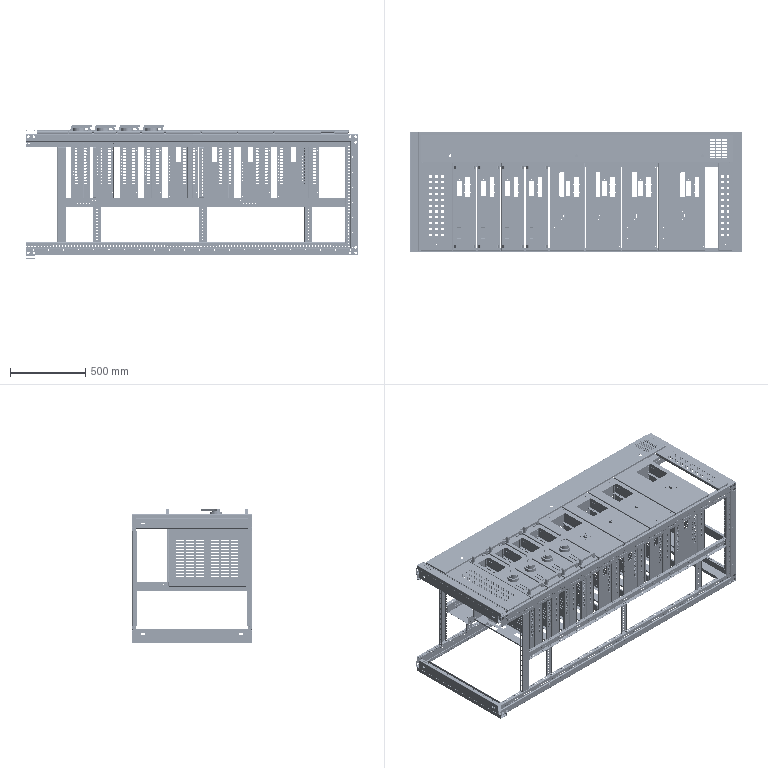Assembly | SolidWorks | mm | 133 component files | 133 solids | 23383 faces | box 2200 x 800 x 893 mm | volume 19032178 mm3 | cylinder 12427 | plane 10700 | spline 216 | torus 40 | commonest cylinder face diameters 5.3 x4638 9.2 x2178 5 x2150 6.5 x956 9 x522 7 x313 1.51 x260 11 x246
Bill of materials:
1.5UnitFrontPanel | 3 |  | Rectangular sheet-type plate with short bent-down flanges on the two long edges. It has a large rectangular cutout with rounded corners near one end, a central round hole with four small holes around it, a small rectangular slot, and small holes spread around the edges.
1.5UnitLeftSidePlate | 3 |  | Tall rectangular thin panel with narrow side flanges. It has one rectangular window, two vertical columns of slots with rounded ends, a row of round holes along one side, scattered holes, and a short stepped or notched area at one end.
1.5UnitRightSidePlate | 3 |  | Tall rectangular thin panel with narrow side flanges. It has one rectangular window, two vertical columns of slots with rounded ends, a row of round holes along one side, scattered holes, and a notched or stepped flange region at the bottom end.
1UnitBackPlate | 8 |  | Long shallow tray-like plate with upturned flanges on all edges. The base has three rectangular cutouts, each with small holes beside it. There are round holes in the end flanges and some side flanges.
DrawerSupport | 12 |  | Long straight channel-type member with a C-shaped cross-section (a web with short return flanges top and bottom). Each end has an end tab with two round holes.
DrawerVentBottomPlate | 8 |  | Rectangular thin panel with short bent flanges on its edges. It has a large grid of horizontal straight slots arranged as six columns (two groups of three) and small holes along the flanges and lower edge.
DrawerWithStretchedHangingAngle | 8 |  | Long channel-type bracket with a C-like cross-section. The web has a rectangular window, four round holes around it, two horizontal slots, and further round holes. One flange edge is interrupted by notches, and the end faces have two round holes.
1855103-DrawerCabinetMiddleColumn | 1 |  | Long, slender, rectangular-section rail with regularly spaced small holes along its faces. The end view shows two round holes and a C-like profile with rounded corners.
1891103-DrawerCabinet | 1 |  | Long, slender, rectangular-section rail with regularly spaced small holes along its faces. The end view shows two larger round holes and a profile with rounded corners.
1UnitFrontPanel | 4 |  | Elongated rectangular plate with shallow bent-down flanges on the long edges. It has a large rectangular cutout with rounded corners near one end, a central round hole with four small holes around it, a small rectangular slot, and small holes around the edges.
1UnitLeftSidePlate | 4 |  | Tall narrow thin panel with narrow side flanges. It has two vertical columns of slots with rounded ends, a row of round holes along one side, scattered holes, and a stepped or notched area at the bottom end.
1UnitRightSidePlate | 4 |  | Tall narrow thin panel with folded side flanges. It has two vertical columns of slots with rounded ends, a row of round holes along one side, and scattered holes. The top end has a flange with chamfered corners that contains two rectangular cutouts.
DrawerControlGateMountingBase-Small | 4 |  | Short, thick-walled cylindrical ring with flat top and bottom faces. It has one small cylindrical boss with a through hole on the inner wall.
DrawerControlGate-Small | 4 |  | Lever-style handle. A cylindrical hub carries a flat arm with a rounded end. Under the hub is a thin circular flange with four radial notches, and below that a short cylindrical spigot.
DrawerGuideRail | 4 |  | Long, narrow, thin strip-like part with small round holes near each end. It has notched or hooked features along one edge and an angled, lobed tab at one end.
DrawerPanelCloseButton | 4 |  | Obround (stadium-shaped) block with a concave saddle-shaped top surface and a smaller rectangular tab projecting from the bottom.
DrawerPanelHandle | 8 |  | Bridge-shaped (U-shaped) bar with a rectangular cross-section. It has a straight top span, two legs that splay slightly outward, and rounded inner and outer corners.
DrawerPanelLabelFrame | 4 |  | Thin, rectangular open frame with straight side members. Both short end members have curved (filleted or coved) inner faces.
MirroredDrawerSlide | 4 |  | Long, narrow, thin strip-like part with small round holes near each end, edge notches or hooks, and an angled tab at one end. It looks like a mirrored counterpart of unnamed part.
2150Column | 1 |  | Long, thin-walled formed channel with a C-shaped profile. One return lip is longer than the other, and the walls carry rows of small holes and elongated slots along the length.
2200CableCompartmentDoor | 1 |  | Long, narrow, thin flat plate with three small round holes along one edge and a grid of small rectangular slots (louvre or vent pattern) near one end.
2200SidePiece | 1 |  | Long rail of thin formed section with a multi-bend profile: flanges, an offset joggle, and a hooked return. Rows of small holes and some larger holes run along the length.
2UnitLeftSidePanel | 1 |  | Rectangular thin panel with narrow flanged edges. It has one rectangular through window, three vertical columns of short slots, and many small round holes along the edges and beside the slot columns.
2UnitPanel | 1 |  | Rectangular thin panel with shallow flanges on its long edges. It has a large rounded-corner rectangular cutout, a central round hole with a four-hole pattern around it, scattered small holes, and a small rectangular slot.
2UnitRightSidePanel | 1 |  | Thin flat rectangular sheet-metal panel with three vertical columns of slotted vents, one rectangular cutout near the upper left, and small round holes around the perimeter and beside the slot columns.
584212VentDoor | 1 |  | Rectangular sheet-metal cover with shallow downturned flanges on its two long sides, three parallel rows of elongated vent slots, and one small round hole near each end.
58492VentDoor | 1 |  | Long, narrow sheet-metal cover with downturned flanges on its long sides, two parallel rows of elongated vent slots, and one small round hole near each end.
740Foot | 1 |  | Long formed sheet-metal channel with a C/U-shaped cross-section, short return lips, and one elongated slot near each end of one side wall.
740Foot-BrowHole | 1 |  | Long formed sheet-metal channel with a C-shaped cross-section, small round holes near each end of the top face, an end tab with a row of small holes, and an elongated slot near each end of the side wall.
740Foot-RearDoorBracket | 1 |  | Long sheet-metal channel with a U-shaped cross-section. One side flange has a long row of evenly spaced round holes, and each end of the other wall has an elongated slot.
800BottomMiddleColumnSupport | 1 |  | Long, slender sheet-metal C-channel with short flanges. Each end of the web has a pair of holes/slots, and there are two small holes near mid-length.
800Brow | 2 |  | Long, closed rectangular hollow section with rounded beads or bulges at two upper corners, a shallow raised strip on the top face, and embossed or engraved lettering on the top surface.
800DrawerCabinetLongSideStop | 3 |  | Elongated sheet-metal bracket with a channel-like profile: a perforated web with a single column of large round holes, and short flanges bent at each end. The top end flange carries two elongated slots.
800DrawerCabinetShortSideStop | 3 |  | Shorter, wider sheet-metal bracket of similar form to unnamed part: a web with a single column of large round holes and short flanges at each end. The top flange carries two small round holes.
800SidePiece | 1 |  | Long formed sheet-metal profile with a multi-bend cross-section (a stepped/offset top segment, a vertical leg and a return), perforated with rows of small round holes along its length and larger holes and notches near the ends.
CableCompartmentPartition | 1 |  | Thin, flat, elongated rectangular plate with a single row of ten evenly spaced large round holes, small rectangular notches along one long edge, and small holes along both long edges.
FrameColumnSupport | 1 |  | Long straight sheet-metal U-channel with an end tab folded across each end. Each end tab has two round holes. The flanges are perforated along their length.
Hinge | 1 |  | Small formed sheet-metal bracket with a Z-shaped joggle. Two rolled cylindrical curls sit at the top edge with a rectangular notch between them. The bracket has three elongated slots.
Mirror1891103-DrawerCabinet1 | 1 |  | Very long, slender rectangular channel or box-section bar. It has dense, regular rows of small perforations along its faces, and the end face or end tab has two round holes.
Mirror2200SidePlate2 | 1 |  | Long sheet-metal rail with a multi-bend open cross-section: a C-shape with an angled joggle in one wall and a return flange. It has a dense row of small holes, a sparser row of holes, larger holes near the ends, and an angled or chamfered end.
Mirror740Foot-BrowHole1 | 1 |  | Sheet-metal channel with a flat web, one tall side wall ending in an inward return lip, and one shorter side wall. A row of round holes runs along the return lip, with elongated slots near each end. The web has two small holes.
Mirror800DrawerCabinetShortSideStop1 | 3 |  | Short sheet-metal C-channel with a tab folded across each end. The top tab has two round holes and the bottom tab has two elongated slots. The web has a single row of 11 equally spaced round holes.
Mirror800SidePlate1 | 1 |  | Medium-length formed sheet-metal rail with a multi-bend profile: an offset web with an angled joggle, side legs, and a return flange. It has rows of small holes along the length, larger holes near the ends, and notched or chamfered ends.
Mirrored2200SidePiece | 1 |  | Long sheet-metal rail with a multi-bend profile: a C-section with an inward lip on one side and an angled joggle leading to an outward bottom flange. It has dense rows of small holes, a sparse row of holes, and larger holes and angled cuts at the ends.
MirrorFrameColumnSupport1 | 1 |  | Long straight sheet-metal U-channel with one folded end tab that has two round holes. One flange has a regular row of round holes along its length.
MirrorMirror2200SidePlate1 | 1 |  | Long sheet-metal rail with a multi-bend profile: a C-section with a lip and an angled joggle leading to a bottom flange. It has dense rows of small holes, a sparse row of holes, and larger end holes with angled end cuts.
Track | 8 |  | Long narrow flat strip with a wider rectangular tab at each end. Each tab has two elongated slots or holes. One end has a raised stepped feature with a rounded, mushroom-like protrusion.
Mates:
1. coincident | 800SidePiece-1 face at (-12.93, 25.557, 400) dir (0, 1, 0) | 2200SidePiece-1 face at (32.07, 25.557, -355) dir (0, 1, 0)
2. coincident | 800SidePiece-1 edge at (29.57, 22.857, -397.5) dir (0, -1, 0) | 2200SidePiece-1 edge at (29.57, -1.743, -397.5) dir (0, 1, 0)
3. coincident | 800SidePiece-1 edge at (-52.93, -4.393, -315) dir (0, 1, 0) | 2200SidePiece-1 edge at (-52.93, -4.393, -315) dir (0, 1, 0)
4. distance | FrameColumnSupport-1 face at (-1962.93, 18.807, -315) dir (-1, 0, 0) | 2200SidePiece-1 edge at (-2167.93, -4.393, -317.5) dir (0, 1, 0)
5. coincident | FrameColumnSupport-1 face at (-1902.93, 18.807, 315) dir (1, 0, 0) | 1891103-DrawerCabinet-1 face at (-1902.93, 20.607, -78) dir (-1, 0, 0)
6. coincident | 800SidePiece-1 edge at (29.57, -1.743, 397.5) dir (0, 1, 0) | Mirrored2200SidePiece-1 edge at (29.57, -1.743, 397.5) dir (0, 1, 0)
7. coincident | 800SidePiece-1 face at (-12.93, 25.557, 400) dir (0, 1, 0) | Mirrored2200SidePiece-1 face at (32.07, 25.557, 355) dir (0, 1, 0)
8. coincident | 800SidePiece-1 edge at (-52.93, -4.393, 315) dir (0, 1, 0) | Mirrored2200SidePiece-1 edge at (-52.93, -4.393, 315) dir (0, 1, 0)
9. coincident | 1891103-DrawerCabinet-1 face at (-1902.93, -4.393, -80) dir (0, -1, 0) | Mirrored2200SidePiece-1 face at (32.07, -4.393, 317.5) dir (0, -1, 0)
10. distance | 2200SidePiece-1 face at (32.07, -4.393, -315) dir (0, 0, 1) | 1891103-DrawerCabinet-1 face at (-1902.93, -2.593, -80) dir (0, 0, -1)
11. coincident | 1891103-DrawerCabinet-1 face at (-1902.93, -2.593, -80) dir (0, 0, -1) | CableCompartmentPartition-1 face at (-1848.644, 2980.948, -80) dir (0, 0, 1)
12. concentric | 1891103-DrawerCabinet-1 edge at (-207.93, 5.607, -80) dir (0, 0, 1) r 2.65 | CableCompartmentPartition-1 edge at (-207.93, 5.607, -80) dir (0, 0, -1) r 4.25
13. parallel | 1891103-DrawerCabinet-1 face at (-1902.93, -2.593, -80) dir (0, 1, 0) | CableCompartmentPartition-1 face at (-1848.644, 13.107, -81.2) dir (0, 1, 0)
14. parallel | 1855103-DrawerCabinetMiddleColumn-1 face at (-50.43, -177.393, -80) dir (0, 1, 0) | Mirrored2200SidePiece-1 face at (32.07, 25.557, 355) dir (0, 1, 0)
15. concentric | CableCompartmentPartition-1 edge at (-207.93, -192.393, -81.2) dir (0, 0, -1) r 4.25 | 1855103-DrawerCabinetMiddleColumn-1 edge at (-207.93, -192.393, -20) dir (0, 0, 1) r 2.65
16. coincident | CableCompartmentPartition-1 face at (-1848.644, 2980.948, -80) dir (0, 0, 1) | 1855103-DrawerCabinetMiddleColumn-1 face at (-1905.43, -200.593, -80) dir (0, 0, -1)
17. concentric | 800DrawerCabinetShortSideStop-1 edge at (-1687.93, 5.607, -80.5) dir (0, 0, 1) r 3.25 | 1891103-DrawerCabinet-1 edge at (-1687.93, 5.607, -80) dir (0, 0, 1) r 2.65
18. concentric | 1891103-DrawerCabinet-1 edge at (-1707.93, 5.607, -80) dir (0, 0, 1) r 2.65 | 800DrawerCabinetShortSideStop-1 edge at (-1707.93, 5.607, -80.5) dir (0, 0, 1) r 3.25
19. distance | 800DrawerCabinetShortSideStop-1 face at (-1675.167, 20.607, -314.5) dir (0, 0, -1) | 2200SidePiece-1 face at (32.07, -4.393, -315) dir (0, 0, 1)
20. concentric | 1891103-DrawerCabinet-1 edge at (-1687.93, 5.607, -20) dir (0, 0, 1) r 2.65 | 800DrawerCabinetLongSideStop-3 edge at (-1687.93, 5.607, -19.5) dir (0, 0, -1) r 3.25
21. concentric | 1891103-DrawerCabinet-1 edge at (-1707.93, 5.607, -20) dir (0, 0, 1) r 2.65 | 800DrawerCabinetLongSideStop-3 edge at (-1707.93, 5.607, -19.5) dir (0, 0, -1) r 3.25
22. distance | 800DrawerCabinetLongSideStop-3 face at (-1675.167, 20.607, -19.5) dir (0, 0, -1) | 1891103-DrawerCabinet-1 face at (-54.93, -2.593, -20) dir (0, 0, 1)
23. coincident | Mirror800SidePlate1-1 edge at (29.57, -771.743, -397.5) dir (0, 1, 0) | Mirror2200SidePlate2-1 edge at (29.57, -747.143, -397.5) dir (0, -1, 0)
24. coincident | Mirror800SidePlate1-1 face at (-12.93, -774.443, 400) dir (0, -1, 0) | Mirror2200SidePlate2-1 face at (32.07, -774.443, -355) dir (0, -1, 0)
25. coincident | Mirror800SidePlate1-1 edge at (-52.93, -744.493, -315) dir (0, -1, 0) | Mirror2200SidePlate2-1 edge at (-52.93, -744.493, -315) dir (0, -1, 0)
26. coincident | Mirror800SidePlate1-1 edge at (29.57, -747.143, 397.5) dir (0, -1, 0) | MirrorMirror2200SidePlate1-1 edge at (29.57, -747.143, 397.5) dir (0, -1, 0)
27. coincident | Mirror800SidePlate1-1 face at (-12.93, -774.443, 400) dir (0, -1, 0) | MirrorMirror2200SidePlate1-1 face at (32.07, -774.443, 355) dir (0, -1, 0)
28. coincident | Mirror800SidePlate1-1 edge at (-52.93, -744.493, 315) dir (0, -1, 0) | MirrorMirror2200SidePlate1-1 edge at (-52.93, -744.493, 315) dir (0, -1, 0)
29. distance | Mirror2200SidePlate2-1 face at (32.07, -744.493, -315) dir (0, 0, 1) | Mirror1891103-DrawerCabinet1-1 face at (-1900.93, -746.293, -80) dir (0, 0, -1)
30. coincident | MirrorFrameColumnSupport1-1 face at (-1960.93, -769.493, -315) dir (0, -1, 0) | MirrorMirror2200SidePlate1-1 face at (32.07, -769.493, 315) dir (0, -1, 0)
31. distance | MirrorFrameColumnSupport1-1 face at (-1960.93, -767.693, -315) dir (-1, 0, 0) | Mirror2200SidePlate2-1 face at (-2167.93, -766.993, -317.7) dir (-1, 0, 0)
32. coincident | Mirror800SidePlate1-1 face at (-50.43, -744.493, 400) dir (0, 1, 0) | Mirror1891103-DrawerCabinet1-1 face at (-1900.93, -744.493, -80) dir (0, 1, 0)
33. coincident | Mirror800SidePlate1-1 face at (-52.93, -744.493, 400) dir (-1, 0, 0) | Mirror1891103-DrawerCabinet1-1 face at (-52.93, -769.493, -22) dir (1, 0, 0)
34. concentric | Mirror1891103-DrawerCabinet1-1 edge at (-1705.93, -754.493, -80) dir (0, 0, -1) r 2.65 | Mirror800DrawerCabinetShortSideStop1-1 face at (-1705.93, -754.493, -82) dir (0, 0, 1) r 3.25
35. concentric | Mirror1891103-DrawerCabinet1-1 edge at (-1685.93, -754.493, -80) dir (0, 0, -1) r 2.65 | Mirror800DrawerCabinetShortSideStop1-1 edge at (-1685.93, -754.493, -80.5) dir (0, 0, -1) r 3.25
36. distance | Mirror800DrawerCabinetShortSideStop1-1 face at (-1718.694, -769.493, -80.5) dir (0, 0, 1) | Mirror1891103-DrawerCabinet1-1 face at (-1900.93, -746.293, -80) dir (0, 0, -1)
37. coincident | 740Foot-BrowHole-1 face at (-2167.93, -4.443, 398.2) dir (-1, 0, 0) | MirrorMirror2200SidePlate1-1 face at (-2167.93, -747.143, 397.3) dir (-1, 0, 0)
38. coincident | 740Foot-BrowHole-1 face at (-2167.93, -744.443, 400) dir (0, 0, 1) | MirrorMirror2200SidePlate1-1 face at (32.07, -774.443, 400) dir (0, 0, 1)
39. coincident | Mirrored2200SidePiece-1 face at (32.07, -4.443, 400) dir (0, -1, 0) | 740Foot-BrowHole-1 face at (-2167.93, -4.443, 333) dir (0, 1, 0)
40. coincident | Mirror2200SidePlate2-1 face at (-2167.93, -747.143, -397.3) dir (-1, 0, 0) | Mirror740Foot-BrowHole1-1 face at (-2167.93, -4.443, -398.2) dir (-1, 0, 0)
41. coincident | Mirror2200SidePlate2-1 face at (32.07, -774.443, -400) dir (0, 0, -1) | Mirror740Foot-BrowHole1-1 face at (-2167.93, -744.443, -400) dir (0, 0, -1)
42. coincident | 2200SidePiece-1 face at (32.07, -4.443, -400) dir (0, -1, 0) | Mirror740Foot-BrowHole1-1 face at (-2082.93, -4.443, -398.2) dir (0, 1, 0)
43. coincident | 740Foot-RearDoorBracket-1 face at (32.07, -4.443, -398.2) dir (1, 0, 0) | 800SidePiece-1 face at (32.07, 25.557, 400) dir (1, 0, 0)
44. coincident | Mirror2200SidePlate2-1 face at (32.07, -774.443, -400) dir (0, 0, -1) | 740Foot-RearDoorBracket-1 face at (32.07, -744.443, -400) dir (0, 0, -1)
45. coincident | 2200SidePiece-1 face at (32.07, -4.443, -400) dir (0, -1, 0) | 740Foot-RearDoorBracket-1 face at (32.07, -4.443, -333) dir (0, 1, 0)
46. coincident | 740Foot-1 face at (32.07, -744.443, 398.2) dir (1, 0, 0) | 800SidePiece-1 face at (32.07, 25.557, 400) dir (1, 0, 0)
47. coincident | MirrorMirror2200SidePlate1-1 face at (32.07, -774.443, 400) dir (0, 0, 1) | 740Foot-1 face at (32.07, -4.443, 400) dir (0, 0, 1)
48. coincident | Mirrored2200SidePiece-1 face at (32.07, -4.443, 400) dir (0, -1, 0) | 740Foot-1 face at (-52.93, -4.443, 398.2) dir (0, 1, 0)
49. coincident | 2150Column-1 face at (-2142.93, -164.443, 400) dir (0, 0, 1) | Mirrored2200SidePiece-1 face at (32.07, 25.557, 400) dir (0, 0, 1)
50. distance | 2150Column-1 face at (7.07, -164.443, 398) dir (0, 1, 0) | Mirrored2200SidePiece-1 face at (32.07, -4.443, 400) dir (0, -1, 0)
51. coincident | 740Foot-1 face at (-52.93, -744.443, 375) dir (-1, 0, 0) | 2150Column-1 face at (-52.93, -143.083, 400) dir (1, 0, 0)
52. concentric | 740Foot-BrowHole-1 edge at (-2137.93, -79.443, 400) dir (0, 0, 1) r 4.25 | 800Brow-1 edge at (-2137.93, -79.443, 400) dir (0, 0, -1) r 6
53. concentric | 740Foot-BrowHole-1 edge at (-2137.93, -669.443, 400) dir (0, 0, 1) r 4.25 | 800Brow-1 edge at (-2137.93, -669.443, 400) dir (0, 0, -1) r 6
54. coincident | 740Foot-BrowHole-1 face at (-2167.93, -744.443, 400) dir (0, 0, 1) | 800Brow-1 face at (-2107.93, 20.557, 400) dir (0, 0, -1)
55. concentric | Mirror740Foot-BrowHole1-1 edge at (-2137.93, -669.443, -400) dir (0, 0, 1) r 4.25 | 800Brow-2 edge at (-2137.93, -669.443, -400) dir (0, 0, 1) r 6
56. concentric | Mirror740Foot-BrowHole1-1 edge at (-2137.93, -79.443, -400) dir (0, 0, 1) r 4.25 | 800Brow-2 edge at (-2137.93, -79.443, -400) dir (0, 0, 1) r 6
57. coincident | 800Brow-2 face at (-2107.93, -769.443, -400) dir (0, 0, 1) | Mirror740Foot-BrowHole1-1 face at (-2167.93, -744.443, -400) dir (0, 0, -1)
58. coincident | 800SidePiece-1 face at (-50.43, -4.393, 400) dir (1, 0, 0) | 800BottomMiddleColumnSupport-1 face at (-50.43, 15.557, -80) dir (-1, 0, 0)
59. coincident | 800BottomMiddleColumnSupport-1 face at (-48.93, -764.443, -20) dir (0, 0, 1) | 1855103-DrawerCabinetMiddleColumn-1 face at (-50.43, -200.593, -20) dir (0, 0, 1)
60. distance | 800BottomMiddleColumnSupport-1 face at (-50.43, 15.557, -20) dir (0, 1, 0) | 800SidePiece-1 face at (-12.93, 25.557, 400) dir (0, 1, 0)
61. coincident | Mirrored2200SidePiece-1 face at (32.07, 18.107, 315) dir (0, -1, 0) | Hinge-1 face at (-1857.93, 18.107, 367.5) dir (0, 1, 0)
62. distance | Hinge-1 face at (-1897.93, -6.993, 370) dir (0, 0, 1) | Mirrored2200SidePiece-1 face at (32.07, -4.443, 375) dir (0, 0, -1)
63. distance | Hinge-1 face at (-1897.93, -6.993, 419.5) dir (-1, 0, 0) | 800Brow-1 face at (-2107.93, 20.557, 425) dir (1, 0, 0)
64. distance | 2200CableCompartmentDoor-1 face at (-2097.93, 10351.309, 119.146) dir (-1, 0, 0) | 800Brow-1 face at (-2107.93, 20.557, 425) dir (1, 0, 0)
65. concentric | Hinge-1 edge at (-1868.93, -1.493, 414) dir (1, 0, 0) r 3 | 2200CableCompartmentDoor-1 face at (-1868.93, -1.493, 414) dir (-1, 0, 0) r 5
66. angle | 2150Column-1 face at (-2142.93, -164.443, 400) dir (0, 0, 1) | 2200CableCompartmentDoor-1 face at (-2097.93, 5.815, 424.798) dir (0, 0.02827, 0.9996)
67. coincident | MirrorMirror2200SidePlate1-1 face at (32.07, -774.443, 400) dir (0, 0, 1) | 584212VentDoor-1 edge at (-1885.93, -764.443, 400) dir (0, 1, 0)
68. distance | 584212VentDoor-1 face at (-2095.675, -764.443, 418.5) dir (0, -1, 0) | MirrorMirror2200SidePlate1-1 face at (32.07, -774.443, 355) dir (0, -1, 0)
69. distance | 584212VentDoor-1 face at (-2097.93, -180.443, 418.5) dir (-1, 0, 0) | 800Brow-1 face at (-2107.93, 20.557, 425) dir (1, 0, 0)
70. coincident | 740Foot-1 face at (32.07, -4.443, 400) dir (0, 0, 1) | 58492VentDoor-1 edge at (-32.93, -764.443, 400) dir (0, 1, 0)
71. distance | 58492VentDoor-1 face at (-122.675, -764.443, 418.5) dir (0, -1, 0) | MirrorMirror2200SidePlate1-1 face at (32.07, -774.443, 355) dir (0, -1, 0)
72. distance | 740Foot-1 face at (32.07, -744.443, 398.2) dir (1, 0, 0) | 58492VentDoor-1 face at (-32.93, -764.443, 418.5) dir (1, 0, 0)
73. coincident | MirrorMirror2200SidePlate1-1 face at (32.07, -744.443, 400) dir (0, 1, 0) | Track-1 face at (-1830.93, -744.443, 387) dir (0, -1, 0)
74. distance | Track-1 face at (-1818.93, -734.443, -47) dir (-1, 0, 0) | MirrorFrameColumnSupport1-1 face at (-1900.93, -767.693, 315) dir (1, 0, 0)
75. distance | Track-1 face at (-1783.93, -739.943, -49) dir (0, 0, -1) | Mirror1891103-DrawerCabinet1-1 face at (-1900.93, -746.293, -80) dir (0, 0, -1)
76. distance | 1UnitDrawer-1/DrawerGuideRail-1 face at (-1787.43, -739.943, -49.5) dir (1, 0, 0) | Track-1 face at (-1786.43, -734.443, 359) dir (-1, 0, 0)
77. distance | MirrorMirror2200SidePlate1-1 face at (32.07, -774.443, 400) dir (0, 0, 1) | 1UnitDrawer-1/1UnitFrontPanel-1 face at (-1730.43, -180.443, 420) dir (0, 0, 1)
78. coincident | Track-1 face at (-1818.93, -739.943, -49) dir (0, 1, 0) | 1UnitDrawer-1/DrawerGuideRail-1 face at (-1815.43, -739.943, 390.5) dir (0, -1, 0)
79. coincident | 1.5UnitDrawer-1/1.5UnitFrontPanel-1 face at (-1240.194, -764.443, 418.5) dir (0, -1, 0) | 1UnitDrawer-4/1UnitFrontPanel-1 face at (-1252.685, -764.443, 406) dir (0, -1, 0)
80. distance | 1.5UnitDrawer-1/1.5UnitFrontPanel-1 face at (-1242.43, -180.443, 418.5) dir (-1, 0, 0) | 1UnitDrawer-4/1UnitFrontPanel-1 face at (-1250.43, -180.443, 400) dir (1, 0, 0)
81. distance | 1.5UnitDrawer-1/1.5UnitFrontPanel-1 face at (-1010.43, -764.443, 420) dir (0, 0, 1) | MirrorMirror2200SidePlate1-1 face at (32.07, -774.443, 400) dir (0, 0, 1)
82. coincident | 2UnitDrawer-1/2UnitPanel-1 face at (-520.194, -764.443, 418.5) dir (0, -1, 0) | 1.5UnitDrawer-3/1.5UnitFrontPanel-1 face at (-760.194, -764.443, 418.5) dir (0, -1, 0)
83. distance | 2UnitDrawer-1/2UnitPanel-1 face at (-522.43, -764.443, 418.5) dir (-1, 0, 0) | 1.5UnitDrawer-3/1.5UnitFrontPanel-1 face at (-530.43, -764.443, 418.5) dir (1, 0, 0)
84. distance | 2UnitDrawer-1/2UnitPanel-1 face at (-522.43, -764.443, 420) dir (0, 0, 1) | MirrorMirror2200SidePlate1-1 face at (32.07, -774.443, 400) dir (0, 0, 1)
85. coincident | DrawerVentBottomPlate-1 face at (221.762, 257.314, -9) dir (0, 0, -1) | DrawerWithStretchedHangingAngle-1 face at (221.762, -120.686, -9) dir (0, 0, -1)
86. distance | DrawerWithStretchedHangingAngle-1 face at (221.762, -120.686, 9) dir (0, 1, 0) | DrawerVentBottomPlate-1 face at (-287.983, -119.686, 9) dir (0, -1, 0)
87. coincident | DrawerVentBottomPlate-1 face at (221.762, -119.686, 9) dir (1, 0, 0) | DrawerWithStretchedHangingAngle-1 face at (221.762, -208.131, 9) dir (1, 0, 0)
88. coincident | DrawerVentBottomPlate-1 edge at (221.762, 190.314, 1) dir (-1, 0, 0) r 3.25 | 1.5UnitLeftSidePlate-2 edge at (221.762, 190.314, 1) dir (1, 0, 0) r 3.25
89. coincident | DrawerVentBottomPlate-1 edge at (221.762, -87.686, 1) dir (-1, 0, 0) r 3.25 | 1.5UnitLeftSidePlate-2 edge at (221.762, -87.686, 1) dir (1, 0, 0) r 3.25
90. coincident | 1.5UnitRightSidePlate-1 edge at (-290.238, -87.686, 1) dir (1, 0, 0) r 3.25 | DrawerVentBottomPlate-1 edge at (-290.238, -87.686, 1) dir (-1, 0, 0) r 3.25
91. coincident | DrawerVentBottomPlate-1 edge at (-290.238, 190.314, 1) dir (-1, 0, 0) r 3.25 | 1.5UnitRightSidePlate-1 edge at (-290.238, 190.314, 1) dir (1, 0, 0) r 3.25
92. coincident | DrawerSupport-2 edge at (221.762, 241.314, 180) dir (1, 0, 0) r 3.25 | 1.5UnitLeftSidePlate-2 edge at (221.762, 241.314, 180) dir (1, 0, 0) r 3.25
93. coincident | 1.5UnitRightSidePlate-1 edge at (-290.238, 221.314, 180) dir (1, 0, 0) r 3.25 | DrawerSupport-2 edge at (-290.238, 221.314, 180) dir (1, 0, 0) r 3.25
94. coincident | 1.5UnitRightSidePlate-1 edge at (-290.238, -173.686, 180) dir (1, 0, 0) r 3.25 | DrawerSupport-3 edge at (-290.238, -173.686, 180) dir (-1, 0, 0) r 3.25
95. coincident | 1.5UnitRightSidePlate-1 edge at (-290.238, -193.686, 180) dir (1, 0, 0) r 3.25 | DrawerSupport-3 edge at (-290.238, -193.686, 180) dir (-1, 0, 0) r 3.25
96. concentric | DrawerVentBottomPlate-1 edge at (45.762, 249.314, -7.5) dir (0, 0, 1) r 3.25 | 1UnitBackPlate-1 edge at (45.762, 249.314, -7.5) dir (0, 0, -1) r 2.65
97. concentric | DrawerVentBottomPlate-1 edge at (-114.238, 249.314, -7.5) dir (0, 0, 1) r 3.25 | 1UnitBackPlate-1 edge at (-114.238, 249.314, -7.5) dir (0, 0, -1) r 2.65
98. coincident | DrawerVentBottomPlate-1 face at (221.762, 257.314, -7.5) dir (0, 0, 1) | 1UnitBackPlate-1 face at (-290.238, 242.314, -7.5) dir (0, 0, -1)
99. coincident | 1.5UnitRightSidePlate-1 face at (-291.738, -210.686, 188.745) dir (0, -1, 0) | 1.5UnitFrontPanel-1 face at (-322.238, -210.686, -25) dir (0, 1, 0)
100. distance | 1.5UnitFrontPanel-1 face at (-322.238, -210.686, -25) dir (0, 0, -1) | DrawerWithStretchedHangingAngle-1 face at (221.762, -120.686, -9) dir (0, 0, -1)
101. distance | 1.5UnitLeftSidePlate-2 face at (233.762, -210.686, -6.745) dir (1, 0, 0) | 1.5UnitFrontPanel-1 face at (261.762, -210.686, 204.763) dir (1, 0, 0)
102. coincident | DrawerVentBottomPlate-1 face at (221.762, 257.314, -9) dir (0, 0, -1) | DrawerWithStretchedHangingAngle-1 face at (221.762, -120.686, -9) dir (0, 0, -1)
103. distance | DrawerWithStretchedHangingAngle-1 face at (221.762, -120.686, 9) dir (0, 1, 0) | DrawerVentBottomPlate-1 face at (-287.983, -119.686, 9) dir (0, -1, 0)
104. coincident | DrawerVentBottomPlate-1 face at (221.762, -119.686, 9) dir (1, 0, 0) | DrawerWithStretchedHangingAngle-1 face at (221.762, -208.131, 9) dir (1, 0, 0)
105. coincident | DrawerVentBottomPlate-1 face at (221.762, -119.686, 9) dir (1, 0, 0) | 1UnitRightSidePlate-1 face at (221.762, 257.314, -9) dir (-1, 0, 0)
106. coincident | 1UnitRightSidePlate-1 face at (223.262, 232.314, -9) dir (0, 0, -1) | DrawerVentBottomPlate-1 face at (221.762, 257.314, -9) dir (0, 0, -1)
107. coincident | DrawerWithStretchedHangingAngle-1 face at (-290.238, -210.686, 1) dir (0, -1, 0) | 1UnitRightSidePlate-1 face at (223.262, -210.686, -6.745) dir (0, -1, 0)
108. coincident | 1UnitLeftSidePlate-1 face at (-302.238, 232.314, -9) dir (0, 0, -1) | DrawerVentBottomPlate-1 face at (221.762, 257.314, -9) dir (0, 0, -1)
109. coincident | DrawerVentBottomPlate-1 face at (-290.238, 232.314, 9) dir (-1, 0, 0) | 1UnitLeftSidePlate-1 face at (-290.238, 257.314, -9) dir (1, 0, 0)
110. coincident | DrawerWithStretchedHangingAngle-1 face at (-290.238, -210.686, 1) dir (0, -1, 0) | 1UnitLeftSidePlate-1 face at (-302.238, -210.686, -6.745) dir (0, -1, 0)
111. coincident | DrawerVentBottomPlate-1 face at (221.762, 257.314, -7.5) dir (0, 0, 1) | 1UnitBackPlate-1 face at (-290.238, 240.314, -7.5) dir (0, 0, -1)
112. coincident | 1UnitBackPlate-1 face at (-290.238, 240.314, 108.245) dir (-1, 0, 0) | 1UnitLeftSidePlate-1 face at (-290.238, 257.314, -9) dir (1, 0, 0)
113. coincident | DrawerVentBottomPlate-1 face at (-290.238, 257.314, -7.5) dir (0, 1, 0) | 1UnitBackPlate-1 face at (-290.238, 257.314, -7.5) dir (0, 1, 0)
114. coincident | DrawerSupport-1 face at (-290.238, -158.686, 111) dir (0, 0, 1) | 1UnitRightSidePlate-1 face at (223.262, -210.686, 111) dir (0, 0, 1)
115. coincident | 1UnitLeftSidePlate-1 edge at (-290.238, -173.686, 100) dir (1, 0, 0) r 3.25 | DrawerSupport-1 edge at (-290.238, -173.686, 100) dir (1, 0, 0) r 3.25
116. distance | 1UnitFrontPanel-1 face at (-322.238, -192.186, 127) dir (0, 0, 1) | DrawerSupport-1 face at (-290.238, -158.686, 111) dir (0, 0, 1)
117. distance | 1UnitFrontPanel-1 face at (-322.238, -198.186, -22.745) dir (-1, 0, 0) | 1UnitLeftSidePlate-1 face at (-302.238, -210.686, -6.745) dir (-1, 0, 0)
118. coincident | 1UnitLeftSidePlate-1 face at (-302.238, -210.686, -6.745) dir (0, -1, 0) | 1UnitFrontPanel-1 face at (261.762, -210.686, -25) dir (0, 1, 0)
119. concentric | 1UnitFrontPanel-1 edge at (-167.238, -212.186, 88) dir (0, -1, 0) r 2.25 | DrawerPanelLabelFrame-1 edge at (-167.238, -212.186, 88) dir (0, 1, 0) r 2.65
120. concentric | 1UnitFrontPanel-1 edge at (-242.238, -212.186, 88) dir (0, -1, 0) r 2.25 | DrawerPanelLabelFrame-1 edge at (-242.238, -212.186, 88) dir (0, 1, 0) r 2.65
121. coincident | 1UnitFrontPanel-1 face at (261.762, -212.186, -25) dir (0, -1, 0) | DrawerPanelLabelFrame-1 face at (-163.738, -212.186, 103) dir (0, 1, 0)
122. concentric | 1UnitFrontPanel-1 edge at (-292.238, -212.186, -14) dir (0, -1, 0) r 2.65 | DrawerPanelHandle-1 edge at (-292.238, -212.186, -14) dir (0, 1, 0) r 3.25
123. coincident | 1UnitFrontPanel-1 face at (261.762, -212.186, -25) dir (0, -1, 0) | DrawerPanelHandle-1 face at (-302.238, -212.186, 106.294) dir (0, 1, 0)
124. parallel | 1UnitFrontPanel-1 face at (-322.238, -192.186, 127) dir (0, 0, 1) | DrawerPanelHandle-1 edge at (-302.238, -212.186, 122.015) dir (1, 0, 0)
125. concentric | 1UnitFrontPanel-1 edge at (231.762, -212.186, -14) dir (0, -1, 0) r 2.65 | DrawerPanelHandle-2 edge at (231.762, -212.186, -14) dir (0, 1, 0) r 3.25
126. coincident | 1UnitFrontPanel-1 face at (261.762, -212.186, -25) dir (0, -1, 0) | DrawerPanelHandle-2 face at (241.762, -212.186, -4.264) dir (0, 1, 0)
127. parallel | 1UnitFrontPanel-1 face at (-322.238, -192.186, 127) dir (0, 0, 1) | DrawerPanelHandle-2 edge at (241.762, -212.186, 122.015) dir (-1, 0, 0)
128. coincident | 1UnitFrontPanel-1 face at (261.762, -212.186, -25) dir (0, -1, 0) | DrawerPanelCloseButton-1 face at (228.512, -212.186, 4.811) dir (0, 1, 0)
129. coincident | 1UnitFrontPanel-1 face at (230.262, -210.686, 23) dir (1, 0, 0) | DrawerPanelCloseButton-1 face at (230.262, -210.186, 17.313) dir (-1, 0, 0)
130. distance | DrawerPanelCloseButton-1 face at (236.762, -210.186, 17.313) dir (0, 0, 1) | 1UnitFrontPanel-1 face at (236.762, -210.686, 23) dir (0, 0, -1)
131. coincident | DrawerGuideRail-1 edge at (-291.738, -152.686, 46) dir (1, 0, 0) r 2.65 | 1UnitLeftSidePlate-1 edge at (-291.738, -152.686, 46) dir (1, 0, 0) r 2.65
132. coincident | 1UnitLeftSidePlate-1 edge at (-291.738, 187.314, 46) dir (1, 0, 0) r 2.65 | DrawerGuideRail-1 edge at (-291.738, 187.314, 46) dir (1, 0, 0) r 2.65
133. coincident | 1UnitRightSidePlate-1 edge at (223.262, 187.314, 46) dir (1, 0, 0) r 2.65 | MirroredDrawerSlide-1 edge at (223.262, 187.314, 46) dir (1, 0, 0) r 2.65
134. coincident | 1UnitRightSidePlate-1 edge at (223.262, -152.686, 46) dir (1, 0, 0) r 2.65 | MirroredDrawerSlide-1 edge at (223.262, -152.686, 46) dir (1, 0, 0) r 2.65
135. concentric | 1UnitFrontPanel-1 edge at (-117.238, -212.186, 36) dir (0, -1, 0) r 3.25 | DrawerControlGateMountingBase-Small-1 edge at (-117.238, -212.186, 36) dir (0, 1, 0) r 2.65
136. concentric | 1UnitFrontPanel-1 edge at (-117.238, -212.186, 36) dir (0, -1, 0) r 3.25 | DrawerControlGateMountingBase-Small-1 edge at (-117.238, -212.186, 36) dir (0, 1, 0) r 2.65
137. concentric | 1UnitFrontPanel-1 edge at (-67.238, -212.186, 36) dir (0, -1, 0) r 3.25 | DrawerControlGateMountingBase-Small-1 edge at (-67.238, -212.186, 36) dir (0, 1, 0) r 2.65
138. coincident | 1UnitFrontPanel-1 face at (261.762, -212.186, -25) dir (0, -1, 0) | DrawerControlGateMountingBase-Small-1 face at (-92.238, -212.186, 61) dir (0, 1, 0)
139. concentric | DrawerControlGateMountingBase-Small-1 face at (-92.238, -212.186, 61) dir (0, -1, 0) r 30 | DrawerControlGate-Small-1 face at (-92.238, -242.186, 61) dir (0, 1, 0) r 28
140. angle | DrawerControlGate-Small-1 face at (-75.588, -257.186, 66.86) dir (0.6266, 0, 0.7793) | 1UnitFrontPanel-1 face at (-322.238, -192.186, 127) dir (0, 0, 1)
141. coincident | DrawerControlGateMountingBase-Small-1 face at (-117.238, -227.186, 36) dir (0, 1, 0) | DrawerControlGate-Small-1 face at (-92.238, -227.186, 61) dir (0, -1, 0)
142. coincident | DrawerVentBottomPlate-1 face at (221.762, 257.314, -9) dir (0, 0, -1) | DrawerWithStretchedHangingAngle-1 face at (221.762, -120.686, -9) dir (0, 0, -1)
143. distance | DrawerWithStretchedHangingAngle-1 face at (221.762, -120.686, 9) dir (0, 1, 0) | DrawerVentBottomPlate-1 face at (-287.983, -119.686, 9) dir (0, -1, 0)
144. coincident | DrawerVentBottomPlate-1 face at (221.762, -119.686, 9) dir (1, 0, 0) | DrawerWithStretchedHangingAngle-1 face at (221.762, -208.131, 9) dir (1, 0, 0)
145. concentric | 2UnitLeftSidePanel-1 edge at (-290.238, -87.686, 1) dir (1, 0, 0) r 3.5 | DrawerVentBottomPlate-1 edge at (-290.238, -87.686, 1) dir (-1, 0, 0) r 3.25
146. concentric | DrawerVentBottomPlate-1 edge at (-290.238, 190.314, 1) dir (-1, 0, 0) r 3.25 | 2UnitLeftSidePanel-1 edge at (-290.238, 190.314, 1) dir (1, 0, 0) r 3.5
147. coincident | DrawerVentBottomPlate-1 face at (-290.238, 232.314, 9) dir (-1, 0, 0) | 2UnitLeftSidePanel-1 face at (-290.238, -210.686, 271) dir (1, 0, 0)
148. concentric | DrawerVentBottomPlate-1 edge at (221.762, -87.686, 1) dir (-1, 0, 0) r 3.25 | 2UnitRightSidePanel-1 edge at (221.762, -87.686, 1) dir (1, 0, 0) r 3.5
149. concentric | DrawerVentBottomPlate-1 edge at (221.762, 190.314, 1) dir (-1, 0, 0) r 3.25 | 2UnitRightSidePanel-1 edge at (221.762, 190.314, 1) dir (1, 0, 0) r 3.5
150. coincident | DrawerVentBottomPlate-1 face at (221.762, -119.686, 9) dir (1, 0, 0) | 2UnitRightSidePanel-1 face at (221.762, -210.686, 271) dir (-1, 0, 0)
151. coincident | DrawerSupport-3 edge at (-290.238, -193.686, 260) dir (-1, 0, 0) r 3.25 | 2UnitLeftSidePanel-1 edge at (-290.238, -193.686, 260) dir (1, 0, 0) r 3.25
152. concentric | DrawerSupport-3 face at (221.762, -173.686, 260) dir (-1, 0, 0) r 3.25 | 2UnitLeftSidePanel-1 face at (-290.238, -173.686, 260) dir (-1, 0, 0) r 3.25
153. coincident | DrawerSupport-2 edge at (-290.238, 221.314, 260) dir (1, 0, 0) r 3.25 | 2UnitLeftSidePanel-1 edge at (-290.238, 221.314, 260) dir (1, 0, 0) r 3.25
154. concentric | DrawerSupport-2 face at (-290.238, 241.314, 260) dir (1, 0, 0) r 3.25 | 2UnitLeftSidePanel-1 face at (-290.238, 241.314, 260) dir (-1, 0, 0) r 3.25
155. coincident | 2UnitLeftSidePanel-1 face at (-291.738, -210.686, 268.745) dir (0, -1, 0) | 2UnitPanel-1 face at (-322.238, -210.686, 287) dir (0, 1, 0)
156. distance | 2UnitPanel-1 face at (261.762, -210.686, -25) dir (0, 0, -1) | DrawerWithStretchedHangingAngle-1 face at (221.762, -120.686, -9) dir (0, 0, -1)
157. distance | 2UnitLeftSidePanel-1 face at (-302.238, -210.686, -6.745) dir (-1, 0, 0) | 2UnitPanel-1 face at (-322.238, -210.686, 284.763) dir (-1, 0, 0)
158. coincident | DrawerVentBottomPlate-1 face at (221.762, 257.314, -7.5) dir (0, 0, 1) | 1UnitBackPlate-1 face at (-290.238, 240.314, -7.5) dir (0, 0, -1)
159. coincident | 1UnitBackPlate-1 face at (221.762, 240.314, -5.245) dir (1, 0, 0) | 2UnitRightSidePanel-1 face at (221.762, -210.686, 271) dir (-1, 0, 0)
160. coincident | DrawerVentBottomPlate-1 face at (-290.238, 257.314, -7.5) dir (0, 1, 0) | 1UnitBackPlate-1 face at (-290.238, 257.314, -7.5) dir (0, 1, 0)